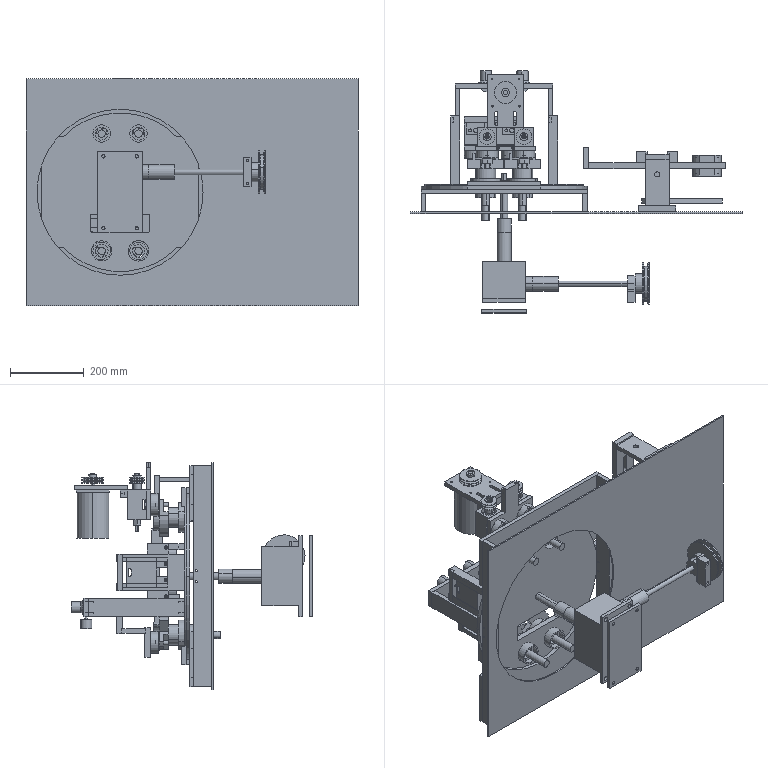Assembly | SolidWorks | mm | 86 component files | 87 solids | 1942 faces | box 900 x 656 x 616.29 mm | volume 16364994 mm3 | cylinder 1056 | plane 736 | cone 150 | commonest cylinder face diameters 5 x140 6.8 x104 7 x102 11 x94 6.6 x82 12 x52 35 x34 15 x28
Bill of materials:
AdjustmentSupportPlate | 2 |  | Long, slender rectangular bar with two small holes drilled into one end face.
AdjustmentTopPlate | 1 |  | Flat rectangular bar or strip plate with six through holes: two larger holes near the middle and two smaller holes at each end.
AdjustmentWheel | 2 |  | Turned part with a short cylindrical shank and a larger head. The head has a short cylindrical rim and a conical taper down to the shank, and a small axial hole in its face.
Axis | 2 |  | Stepped, hollow cylindrical part with a central bore running the full length. It has several diameter steps, a larger collar with flats near one end, and a short, slightly tapered spigot at that end.
BearingHeighteningSeat | 1 |  | Rectangular block, tall compared with its width, with two through holes across its thinner dimension near each end.
BearingHousing1 | 2 |  | Tubular sleeve with a large through bore and a raised flange around its middle. The flange has three equally spaced through holes.
BearingHousing2 | 2 |  | Flanged bushing: a cylindrical hub with a wider flange at one end, a large central through bore, and three equally spaced holes in the flange.
BearingHousingMountingPlate | 2 |  | Long flat rectangular bar with through holes of different sizes: one small hole, one medium hole, and near one end a large hole surrounded by four small holes in a square pattern. Two holes are drilled into the end face nearest the large hole.
BevelGearPlate1 | 1 |  | Thick rectangular plate with many through holes: four in a row along one edge, two larger holes in the middle, and five along the opposite edge. A shallow step or groove runs along one long edge on one face.
BevelGearPlate2 | 2 |  | Solid rectangular block with three vertical through holes in a row: a larger centre hole between two smaller holes, offset toward one long side.
BrassGuideRail | 2 |  | Thick rectangular plate with an undercut channel (T-slot-like profile) along one edge, four blind holes with conical bottoms, and one central through hole on the main face.
CenterAxis | 1 |  | Solid stepped round shaft: a long main diameter, a reduced-diameter section at one end, and two successive smaller steps at the other end.
Coupling1 | 1 |  | Thick-walled cylindrical sleeve with a central through bore that has a single rectangular keyway, plus two small holes on the outer cylindrical surface near each end.
Coupling2 | 1 |  | Solid cylindrical hub or sleeve with a smaller central through bore that has one rectangular keyway; plain outer surface.
CouplingAxis | 4 |  | Solid stepped round shaft or pin with four coaxial diameter sections: a long small-diameter end, a short largest-diameter collar, a middle step, and a slightly smaller end section.
CouplingPlate | 1 |  | Flat inverted-T plate: a wide rectangular base with a narrower rectangular tab rising from its center. The base has two large circular through holes, each surrounded by eight small holes on a bolt circle. Two small holes go into the top edge of the tab.
Disc | 1 |  | Thin circular disc with four large circular through holes (two near the top, two slightly larger near the bottom), a small central hole, and a rounded-corner rectangular slot below the center. The edge views show a slight step around the rim.
DiscBasePlate | 1 |  | Two separate thin rectangular plates under a single ID, placed mirrored with a gap between them. Each has a large circular-arc cutout on its inner long edge, so together they outline a circular opening. Each plate has small holes near its corners and near the ends of the arc.
DiscLimitPlate | 2 |  | Thick rectangular bar with a shallow concave circular-arc cut along one long edge, so it is narrowest at mid-length. There are two through holes near the ends along the straight edge.
DiscLimitPlateBasePlate | 2 |  | Straight rectangular bar with two circular through holes, one near each end, through the narrow dimension.
HolePunchingCouplingBushing | 1 |  | Plain thick-walled cylindrical tube or spacer with a concentric round through bore, about as long as its diameter.
Die | 2 |  | Rectangular block with an obround slot through its thickness near one edge, and a narrow channel running from that edge into the slot.
LocatingDieAdjustmentBlock | 2 |  | Elongated stepped block: a thinner full-length flange plate with a small hole at each end, joined to a thicker shorter central body. A larger circular through hole passes through the middle.
LocatingDieHolder | 2 |  | U-shaped (C-shaped) flat frame plate: a solid back section with two parallel arms around a large rectangular opening that is open at one end. Small rectangular notches cut into one face near the free ends of the arms.
LockingWheel | 2 |  | Coaxial stepped cylinder: a large short cylindrical base, then a short medium-diameter step, then a long slender pin.
LowerRollerFixingRing | 4 |  | Thick circular disc with a large central through hole and four smaller through holes evenly spaced on a circle around it.
Motor | 1 |  | Cylindrical body topped by a thin square plate with four corner holes, and a slender cylindrical shaft sticking out of the plate's centre.
Motor2 | 1 |  | Rectangular box-shaped body with a thin rectangular flange plate on one face that has four corner holes. A cylindrical boss with a smaller shaft sticks out of a side face.
MotorMount | 1 |  | Flat rectangular plate with one large round through hole, four small round holes arranged in a rectangle, and two parallel elongated slots.
MotorMount2 | 1 |  | Thin flat rectangular plate with four small round through holes near the corners.
MotorPlateFixingBlock | 1 |  | Rectangular bar block with two larger through holes along one axis, through the side faces, and two smaller through holes at right angles to them, through the top face.
MotorPulley | 1 |  | Round grooved wheel with two V-shaped circumferential grooves, a raised cylindrical hub on one face, a central through bore, and small radial holes in the hub.
p002 | 1 |  | Extruded profile part: a straight rectangular bar with a lug off one side that has a semicircular end and a round through hole.
Panel | 1 |  | Very thin rectangular sheet with one large circular hole set toward one end.
PunchingAxisSeat | 2 |  | Rectangular block with a large stepped/counterbored round bore from the top, a rectangular notch or slot cut across one side, and four round holes in a side face.
RearRoller | 2 |  | Shaft with a disc on one end. The disc has a wedge-shaped sector cut out, and a narrower arm with a round hole extends into that cut-out area. A short cylindrical boss is on the opposite face.
ReducerCoupling | 1 |  | Long slender stepped cylindrical shaft: larger-diameter central body with a shorter, reduced-diameter journal at each end.
ReducerPulley | 1 |  | Single-groove sheave/pulley-like disc with a cylindrical hub on one side and a central bore with a keyway notch.
Roller | 2 |  | Semicircular (half-disc) body with a rectangular upright tab that has a round hole, a long cylindrical pin sticking out of one face, and a short cylindrical boss on the opposite face.
SmallPulley | 2 |  | Double-groove V-pulley-like body with three flanges forming two V-grooves, a cylindrical hub extending on both sides, and a keyed central bore.
SpringPullPlate | 1 |  | Flat L-shaped plate of constant thickness with four through-holes: one larger and two small holes in the short leg, and one medium hole near the end of the long leg.
SpringPullPlateFixingAxis | 1 |  | Stepped cylindrical pin: a short larger-diameter cylindrical head with a longer, smaller-diameter plain shank.
SupportPlate_2 | 1 |  | Thick rectangular plate with two large circular through-bores. Each bore is surrounded by four small holes in a square pattern, and a row of five holes runs along the upper edge. One edge has a rectangular step or rebate.
SupportPlate | 2 |  | Long, thin rectangular bar or strip with a few small holes on its narrow faces: pairs near each end on one face and two holes near mid-length on the adjacent face.
SupportPlate2 | 1 |  | Rectangular flat plate or block with five evenly spaced round holes drilled into one long edge face.
TractionBasePlate | 1 |  | Long, flat rectangular plate with four corner holes, two pairs of smaller holes (one pair near each end region), and one single hole lower down the centreline.
TractionBearingHousing | 4 |  | Round flange with two parallel flats, a large central bore, four through-holes at the corners, and a raised annular pilot boss on one face.
TractionHandwheelAdjustmentPlate | 1 |  | Solid rectangular block with one round through-hole perpendicular to its largest face.
TractionSmallCylinderSeat | 1 |  | Plain rectangular block with a roughly square footprint. Its height is less than its width. No holes, cutouts, chamfers or other features are visible.
TractionTensionPlate | 2 |  | Thick rectangular plate, close to square in face view. It has two round through-holes lined up along one edge and one horizontal obround (slotted) through-hole near the opposite edge.
TractionUpperPlate | 1 |  | Long, narrow, thin flat bar. Along its centerline it has three elongated through-slots of different lengths and widths, plus one larger round hole near one end. It also has four small round holes, two near each end.
TractionVerticalPlate | 2 |  | Rectangular flat plate with one round hole through the top face, set off-center toward one end. Two smaller round holes are drilled into one long side face.
TurntableFixingNut | 4 |  | Cylindrical sleeve or bushing with a concentric round central bore through its length. Four evenly spaced rectangular notches run lengthwise along the full length of the outer surface.
Mates:
1. coincident | Panel-1 face at (-419.784, 370.983, 311.5) dir (0, 1, 0) | SupportPlate-1 face at (-389.784, 370.983, 304) dir (0, -1, 0)
2. concentric | DiscBasePlate-1 face at (-164.784, 430.983, 4) dir (0, -1, 0) r 215 | Panel-1 face at (-164.784, 370.983, 4) dir (0, -1, 0) r 225
3. distance | DiscBasePlate-1 face at (-164.784, 420.983, 4) dir (0, -1, 0) | Panel-1 face at (-419.784, 370.983, 311.5) dir (0, 1, 0)
4. coincident | DiscBasePlate-1 face at (-389.784, 430.983, 154) dir (-1, 0, 0) | SupportPlate-1 face at (-389.784, 420.983, 304) dir (-1, 0, 0)
5. coincident | DiscBasePlate-1 face at (60.216, 430.983, 304) dir (0, 0, 1) | SupportPlate-1 face at (-389.784, 370.983, 304) dir (0, 0, 1)
6. coincident | DiscBasePlate-1 face at (60.216, 430.983, 304) dir (0, 0, 1) | SupportPlate-2 face at (48.216, 370.983, 304) dir (0, 0, 1)
7. coincident | DiscBasePlate-1 face at (60.216, 430.983, 154) dir (1, 0, 0) | SupportPlate-2 face at (60.216, 420.983, 304) dir (1, 0, 0)
8. coincident | Panel-1 face at (-419.784, 370.983, 311.5) dir (0, 1, 0) | SupportPlate-2 face at (48.216, 370.983, 304) dir (0, -1, 0)
9. concentric | DiscBasePlate-1 face at (-164.784, 430.983, 4) dir (0, -1, 0) r 215 | Disc-1 face at (-164.784, 445.983, 4) dir (0, -1, 0) r 225
10. coincident | Disc-1 face at (-164.784, 430.983, 4) dir (0, -1, 0) | DiscBasePlate-1 face at (-164.784, 430.983, 4) dir (0, 1, 0)
11. parallel | DiscBasePlate-1 face at (60.216, 430.983, -296) dir (0, 0, -1) | Disc-1 face at (-239.784, 445.983, -105.5) dir (0, 0, 1)
12. concentric | Disc-1 face at (-164.784, 440.983, 4) dir (0, 1, 0) r 215 | DiscLimitPlate-1 face at (-164.784, 452.983, 4) dir (0, -1, 0) r 215
13. coincident | DiscLimitPlate-1 face at (-164.784, 440.983, 4) dir (0, -1, 0) | Disc-1 face at (-164.784, 440.983, 4) dir (0, 1, 0)
14. parallel | DiscBasePlate-1 face at (60.216, 430.983, 304) dir (0, 0, 1) | DiscLimitPlate-1 face at (-264.784, 452.983, 244.329) dir (0, 0, 1)
15. coincident | DiscBasePlate-1 face at (-164.784, 430.983, 4) dir (0, 1, 0) | DiscLimitPlateBasePlate-1 face at (-264.784, 430.983, 229.329) dir (0, -1, 0)
16. coincident | DiscLimitPlate-1 face at (-264.784, 452.983, 194.329) dir (-1, 0, 0) | DiscLimitPlateBasePlate-1 face at (-264.784, 430.983, 244.329) dir (-1, 0, 0)
17. coincident | DiscLimitPlate-1 face at (-264.784, 452.983, 244.329) dir (0, 0, 1) | DiscLimitPlateBasePlate-1 face at (-264.784, 430.983, 244.329) dir (0, 0, 1)
18. concentric | Disc-1 face at (-164.784, 440.983, 4) dir (0, 1, 0) r 215 | DiscLimitPlate-2 face at (-164.784, 452.983, 4) dir (0, -1, 0) r 215
19. parallel | DiscBasePlate-1 face at (60.216, 430.983, -296) dir (0, 0, -1) | DiscLimitPlate-2 face at (-64.784, 452.983, -236.329) dir (0, 0, -1)
20. coincident | DiscLimitPlate-2 face at (-164.784, 440.983, 4) dir (0, -1, 0) | Disc-1 face at (-164.784, 440.983, 4) dir (0, 1, 0)
21. coincident | DiscBasePlate-1 face at (-164.784, 430.983, 4) dir (0, 1, 0) | DiscLimitPlateBasePlate-2 face at (-264.784, 430.983, -221.329) dir (0, -1, 0)
22. coincident | DiscLimitPlate-2 face at (-64.784, 452.983, -186.329) dir (1, 0, 0) | DiscLimitPlateBasePlate-2 face at (-64.784, 440.983, -236.329) dir (1, 0, 0)
23. coincident | DiscLimitPlate-2 face at (-64.784, 452.983, -236.329) dir (0, 0, -1) | DiscLimitPlateBasePlate-2 face at (-264.784, 440.983, -236.329) dir (0, 0, -1)
24. coincident | Disc-1 face at (-164.784, 445.983, 4) dir (0, 1, 0) | AdjustmentSupportPlate-1 face at (-285.284, 445.983, -105.5) dir (0, -1, 0)
25. parallel | Disc-1 face at (-84.784, 445.983, -100.5) dir (-1, 0, 0) | AdjustmentSupportPlate-1 face at (-285.284, 705.983, -55.5) dir (1, 0, 0)
26. coincident | Disc-1 face at (-239.784, 445.983, -105.5) dir (0, 0, 1) | AdjustmentSupportPlate-1 face at (-285.284, 705.983, -105.5) dir (0, 0, -1)
27. coincident | Disc-1 face at (-164.784, 445.983, 4) dir (0, 1, 0) | AdjustmentSupportPlate-2 face at (-32.284, 445.983, -55.5) dir (0, -1, 0)
28. coincident | AdjustmentSupportPlate-1 face at (-285.284, 705.983, -55.5) dir (0, 0, 1) | AdjustmentSupportPlate-2 face at (-32.284, 445.983, -55.5) dir (0, 0, 1)
29. distance | AdjustmentSupportPlate-2 face at (-32.284, 445.983, -105.5) dir (1, 0, 0) | AdjustmentSupportPlate-1 face at (-297.284, 705.983, -55.5) dir (-1, 0, 0)
30. coincident | AdjustmentTopPlate-1 face at (-297.284, 705.983, -105.5) dir (0, -1, 0) | AdjustmentSupportPlate-1 face at (-285.284, 705.983, -105.5) dir (0, 1, 0)
31. coincident | AdjustmentTopPlate-1 face at (-297.284, 705.983, -55.5) dir (-1, 0, 0) | AdjustmentSupportPlate-1 face at (-297.284, 705.983, -55.5) dir (-1, 0, 0)
32. coincident | AdjustmentTopPlate-1 face at (-297.284, 705.983, -55.5) dir (0, 0, 1) | AdjustmentSupportPlate-1 face at (-285.284, 705.983, -55.5) dir (0, 0, 1)
33. distance | Disc-1 face at (-244.784, 445.983, -60.5) dir (1, 0, 0) | AdjustmentSupportPlate-1 face at (-285.284, 705.983, -55.5) dir (1, 0, 0)
34. concentric | Disc-1 edge at (-214.784, 445.983, 163) dir (0, -1, 0) r 23.5 | BearingHousing2-1 face at (-214.784, 440.309, 163) dir (0, -1, 0) r 40
35. coincident | Disc-1 face at (-164.784, 445.983, 4) dir (0, 1, 0) | BearingHousing2-1 face at (-250.623, 445.983, 180.764) dir (0, -1, 0)
36. concentric | Disc-1 face at (-214.784, 445.983, -155) dir (0, -1, 0) r 27.5 | BearingHousing1-1 face at (-214.784, 440.309, -155) dir (0, -1, 0) r 27.5
37. coincident | Disc-1 face at (-164.784, 445.983, 4) dir (0, 1, 0) | BearingHousing1-1 face at (-249.957, 445.983, -174.049) dir (0, -1, 0)
38. concentric | Disc-1 face at (-114.784, 445.983, 163) dir (0, -1, 0) r 23.5 | BearingHousing2-2 face at (-114.784, 440.309, 163) dir (0, -1, 0) r 40
39. coincident | Disc-1 face at (-164.784, 445.983, 4) dir (0, 1, 0) | BearingHousing2-2 face at (-150.95, 445.983, 145.912) dir (0, -1, 0)
40. concentric | Disc-1 face at (-114.784, 445.983, -155) dir (0, -1, 0) r 27.5 | BearingHousing1-2 face at (-114.784, 440.309, -155) dir (0, -1, 0) r 27.5
41. coincident | Disc-1 face at (-164.784, 445.983, 4) dir (0, 1, 0) | BearingHousing1-2 face at (-142.56, 445.983, -183.783) dir (0, -1, 0)
42. concentric | BearingHousing1-2 face at (-114.784, 440.309, -155) dir (0, -1, 0) r 17.5 | RearRoller-3 face at (-114.784, 404.838, -155) dir (0, -1, 0) r 10
43. concentric | BearingHousing1-1 face at (-214.784, 440.309, -155) dir (0, -1, 0) r 17.5 | RearRoller-4 face at (-214.784, 404.838, -155) dir (0, -1, 0) r 10
44. parallel | RearRoller-3 face at (-151.129, 348.983, -199.045) dir (0.6062, 0, -0.7953) | RearRoller-4 face at (-251.129, 348.983, -199.045) dir (0.6062, 0, -0.7953)
45. coincident | RearRoller-3 face at (-93.568, 513.983, -182.837) dir (0, 1, 0) | RearRoller-4 face at (-193.568, 513.983, -182.837) dir (0, 1, 0)
46. concentric | BearingHousing2-1 face at (-214.784, 440.309, 163) dir (0, -1, 0) r 17.5 | Roller-5 face at (-214.784, 444.838, 163) dir (0, -1, 0) r 10
47. coincident | BearingHousing2-1 face at (-235.839, 488.983, 173.436) dir (0, 1, 0) | Roller-5 face at (-264.482, 488.983, 168.486) dir (0, -1, 0)
48. concentric | BearingHousing2-2 face at (-114.784, 440.309, 163) dir (0, -1, 0) r 17.5 | Roller-6 face at (-114.784, 444.838, 163) dir (0, -1, 0) r 10
49. coincident | BearingHousing2-2 face at (-136.031, 488.983, 152.961) dir (0, 1, 0) | Roller-6 face at (-164.482, 488.983, 168.486) dir (0, -1, 0)
50. parallel | Roller-5 face at (-195.761, 388.983, 216.843) dir (0.994, 0, -0.1097) | Roller-6 face at (-95.761, 388.983, 216.843) dir (0.994, 0, -0.1097)
51. coincident | RearRoller-3 face at (-84.476, 488.983, -194.767) dir (0, -1, 0) | RearRoller-4 face at (-184.476, 488.983, -194.767) dir (0, -1, 0)
52. coincident | BearingHousing1-1 face at (-235.448, 488.983, -166.191) dir (0, 1, 0) | RearRoller-4 face at (-184.476, 488.983, -194.767) dir (0, -1, 0)
53. concentric | Roller-5 face at (-210.944, 388.983, 197.789) dir (0, 1, 0) r 6 | CouplingAxis-1 face at (-210.944, 520.733, 197.789) dir (0, 1, 0) r 6
54. concentric | LowerRollerFixingRing-1 face at (-210.944, 542.523, 197.789) dir (0, 1, 0) r 10 | CouplingAxis-1 face at (-210.944, 520.733, 197.789) dir (0, 1, 0) r 6
55. coincident | LowerRollerFixingRing-1 face at (-193.444, 525.983, 197.789) dir (0, 1, 0) | CouplingAxis-1 edge at (-210.944, 525.983, 197.789) dir (0, 1, 0) r 7.5
56. concentric | CouplingPlate-1 face at (-210.944, 548.983, 197.789) dir (0, -1, 0) r 17.5 | CouplingAxis-1 face at (-210.944, 520.733, 197.789) dir (0, 1, 0) r 7
57. parallel | DiscLimitPlateBasePlate-1 face at (-264.784, 430.983, 244.329) dir (0, 0, 1) | CouplingPlate-1 face at (-135.944, 548.983, 312.789) dir (0, 0, 1)
58. concentric | CouplingPlate-1 face at (-210.944, 548.983, 220.789) dir (0, 1, 0) r 2.5 | LowerRollerFixingRing-1 face at (-210.944, 516.983, 220.789) dir (0, -1, 0) r 3.3
59. concentric | CouplingPlate-1 face at (-233.944, 548.983, 197.789) dir (0, 1, 0) r 2.5 | LowerRollerFixingRing-1 face at (-233.944, 516.983, 197.789) dir (0, -1, 0) r 3.3
60. coincident | CouplingPlate-1 face at (-79.944, 536.983, 237.789) dir (0, -1, 0) | LowerRollerFixingRing-1 face at (-180.944, 536.983, 197.789) dir (0, 1, 0)
61. coincident | Roller-5 face at (-249.572, 513.983, 166.84) dir (0, 1, 0) | CouplingAxis-1 face at (-215.967, 513.983, 194.507) dir (0, -1, 0)
62. concentric | CouplingPlate-1 face at (-110.944, 548.983, 197.789) dir (0, -1, 0) r 17.5 | CouplingAxis-2 face at (-110.944, 520.733, 197.789) dir (0, 1, 0) r 7
63. concentric | CouplingPlate-1 face at (-110.944, 548.983, 197.789) dir (0, -1, 0) r 17.5 | LowerRollerFixingRing-2 face at (-110.944, 542.523, 197.789) dir (0, 1, 0) r 17.5
64. coincident | CouplingPlate-1 face at (-79.944, 536.983, 237.789) dir (0, -1, 0) | LowerRollerFixingRing-2 face at (-80.944, 536.983, 197.789) dir (0, 1, 0)
65. concentric | CouplingPlate-1 face at (-110.944, 548.983, 220.789) dir (0, 1, 0) r 2.5 | LowerRollerFixingRing-2 face at (-110.944, 516.983, 220.789) dir (0, -1, 0) r 5.5
66. coincident | Roller-6 face at (-149.572, 513.983, 166.84) dir (0, 1, 0) | CouplingAxis-2 face at (-113.911, 513.983, 192.574) dir (0, -1, 0)
67. coincident | CouplingPlate-1 face at (-241.944, 548.983, 157.789) dir (0, 0, -1) | PunchingAxisSeat-1 face at (-185.944, 598.983, 157.789) dir (0, 0, -1)
68. coincident | CouplingPlate-1 face at (-79.944, 548.983, 237.789) dir (0, 1, 0) | PunchingAxisSeat-1 face at (-185.944, 548.983, 237.789) dir (0, -1, 0)
69. concentric | CouplingPlate-1 edge at (-226.944, 548.983, 217.789) dir (0, 1, 0) r 2.5 | PunchingAxisSeat-1 edge at (-226.944, 598.983, 217.789) dir (0, 1, 0) r 3.5
70. coincident | CouplingPlate-1 face at (-79.944, 548.983, 237.789) dir (0, 0, 1) | PunchingAxisSeat-2 face at (-85.944, 598.983, 237.789) dir (0, 0, 1)
71. coincident | CouplingPlate-1 face at (-79.944, 548.983, 237.789) dir (0, 1, 0) | PunchingAxisSeat-2 face at (-85.944, 548.983, 237.789) dir (0, -1, 0)
72. concentric | CouplingPlate-1 edge at (-94.944, 548.983, 177.789) dir (0, 1, 0) r 2.5 | PunchingAxisSeat-2 face at (-94.944, 548.983, 177.789) dir (0, 1, 0) r 3.5
73. coincident | MotorPlateFixingBlock-1 face at (-110.944, 598.983, 217.789) dir (0, -1, 0) | PunchingAxisSeat-2 face at (-85.944, 598.983, 237.789) dir (0, 1, 0)
74. concentric | CouplingAxis-3 face at (-242.621, 520.733, -176.215) dir (0, 1, 0) r 6 | LowerRollerFixingRing-4 face at (-242.621, 542.523, -176.215) dir (0, 1, 0) r 10
75. coincident | CouplingAxis-3 face at (-233.626, 525.983, -175.907) dir (0, 1, 0) | LowerRollerFixingRing-4 face at (-260.013, 525.983, -174.275) dir (0, 1, 0)
76. concentric | RearRoller-4 face at (-242.621, 348.983, -176.215) dir (0, 1, 0) r 6 | CouplingAxis-3 face at (-242.621, 520.733, -176.215) dir (0, 1, 0) r 6
77. coincident | RearRoller-4 face at (-193.568, 513.983, -182.837) dir (0, 1, 0) | CouplingAxis-3 face at (-236.624, 513.983, -176.01) dir (0, -1, 0)
78. coincident | LowerRollerFixingRing-5 face at (-154.995, 525.983, -163.841) dir (0, 1, 0) | CouplingAxis-5 face at (-134.193, 525.983, -173.059) dir (0, 1, 0)
79. concentric | LowerRollerFixingRing-5 face at (-142.621, 542.523, -176.215) dir (0, 1, 0) r 17.5 | CouplingAxis-5 face at (-142.621, 520.733, -176.215) dir (0, 1, 0) r 7
80. concentric | RearRoller-3 face at (-142.621, 348.983, -176.215) dir (0, 1, 0) r 6 | CouplingAxis-5 face at (-142.621, 520.733, -176.215) dir (0, 1, 0) r 6
81. coincident | RearRoller-3 face at (-93.568, 513.983, -182.837) dir (0, 1, 0) | CouplingAxis-5 face at (-137.002, 513.983, -174.111) dir (0, -1, 0)
82. coincident | LowerRollerFixingRing-4 face at (-272.436, 536.983, -172.888) dir (0, 1, 0) | SupportPlate_2-1 face at (-112.621, 536.983, -216.215) dir (0, -1, 0)
83. concentric | SupportPlate_2-1 face at (-242.621, 552.983, -176.215) dir (0, -1, 0) r 17.5 | CouplingAxis-3 face at (-242.621, 520.733, -176.215) dir (0, 1, 0) r 7
84. concentric | LowerRollerFixingRing-5 face at (-126.357, 516.983, -192.479) dir (0, -1, 0) r 3.3 | SupportPlate_2-1 edge at (-126.357, 552.983, -192.479) dir (0, 1, 0) r 2.5
85. concentric | SupportPlate_2-1 edge at (-252.621, 550.983, -144.215) dir (0, 1, 0) r 3.3 | SupportPlate2-3 edge at (-252.621, 550.983, -144.215) dir (0, -1, 0) r 3.4
86. concentric | SupportPlate_2-1 edge at (-132.621, 550.983, -144.215) dir (0, 1, 0) r 3.3 | SupportPlate2-3 edge at (-132.621, 550.983, -144.215) dir (0, -1, 0) r 3.4
87. parallel | SupportPlate2-3 face at (-272.621, 614.983, -138.215) dir (0, 1, 0) | BevelGearPlate1-2 face at (-112.621, 614.983, -138.215) dir (0, -1, 0)
88. concentric | SupportPlate2-3 face at (-132.621, 614.983, -144.215) dir (0, 1, 0) r 3.4 | BevelGearPlate1-2 edge at (-132.621, 628.983, -144.215) dir (0, -1, 0) r 3.5
89. concentric | SupportPlate2-3 face at (-132.621, 614.983, -144.215) dir (0, 1, 0) r 3.4 | BevelGearPlate1-2 edge at (-132.621, 628.983, -144.215) dir (0, -1, 0) r 3.5
90. concentric | SupportPlate2-3 face at (-252.621, 614.983, -144.215) dir (0, 1, 0) r 3.4 | BevelGearPlate1-2 face at (-252.621, 612.983, -144.215) dir (0, 1, 0) r 3.5
91. coincident | SupportPlate2-3 face at (-272.621, 614.983, -138.215) dir (0, 1, 0) | BevelGearPlate1-2 edge at (-112.621, 614.983, -150.215) dir (0, 0, 1)
92. concentric | SupportPlate_2-1 face at (-142.621, 552.983, -176.215) dir (0, -1, 0) r 17.5 | LowerRollerFixingRing-5 edge at (-142.621, 536.983, -176.215) dir (0, 1, 0) r 17.5
93. concentric | SupportPlate_2-1 face at (-126.357, 552.983, -192.479) dir (0, 1, 0) r 2.5 | LowerRollerFixingRing-5 face at (-126.357, 516.983, -192.479) dir (0, -1, 0) r 5.5
94. concentric | BevelGearPlate1-2 face at (-257.621, 628.983, -79.715) dir (0, 1, 0) r 5.5 | BevelGearPlate2-1 face at (-257.621, 612.983, -79.715) dir (0, 1, 0) r 3.4
95. coincident | BevelGearPlate1-2 face at (-112.621, 612.983, -67.215) dir (0, -1, 0) | BevelGearPlate2-1 face at (-266.621, 612.983, -67.215) dir (0, 1, 0)
96. parallel | BevelGearPlate1-2 face at (-112.621, 612.983, -67.215) dir (0, 0, 1) | BevelGearPlate2-1 face at (-266.621, 580.983, -67.215) dir (0, 0, 1)
97. coincident | SupportPlate_2-1 face at (-112.621, 550.983, -150.215) dir (0, 1, 0) | SupportPlate2-3 face at (-272.621, 550.983, -138.215) dir (0, -1, 0)
98. concentric | BevelGearPlate1-2 face at (-159.621, 628.983, -79.715) dir (0, 1, 0) r 5.5 | BevelGearPlate2-2 face at (-159.621, 612.983, -79.715) dir (0, 1, 0) r 3.4
99. coincident | BevelGearPlate1-2 face at (-112.621, 612.983, -67.215) dir (0, 0, 1) | BevelGearPlate2-2 face at (-168.621, 580.983, -67.215) dir (0, 0, 1)
100. coincident | BevelGearPlate1-2 face at (-112.621, 612.983, -67.215) dir (0, -1, 0) | BevelGearPlate2-2 face at (-168.621, 612.983, -67.215) dir (0, 1, 0)
101. concentric | PunchingAxisSeat-1 face at (-210.944, 573.983, 237.789) dir (0, 0, -1) r 11 | Axis-1 face at (-210.944, 573.983, 177.508) dir (0, 0, 1) r 7
102. coincident | PunchingAxisSeat-1 face at (-185.944, 598.983, 157.789) dir (0, 0, -1) | Axis-1 face at (-219.435, 579.265, 157.789) dir (0, 0, 1)
103. concentric | PunchingAxisSeat-2 face at (-110.944, 573.983, 225.789) dir (0, 0, 1) r 20 | Axis-2 face at (-110.944, 573.983, 177.508) dir (0, 0, 1) r 7
104. coincident | PunchingAxisSeat-2 face at (-85.944, 598.983, 157.789) dir (0, 0, -1) | Axis-2 face at (-102.626, 579.535, 157.789) dir (0, 0, 1)
105. parallel | Axis-1 face at (-216.039, 577.152, 282.789) dir (0, 0, 1) | SmallPulley-1 face at (-189.444, 573.983, 255.789) dir (0, 0, -1)
106. coincident | PunchingAxisSeat-1 face at (-185.944, 598.983, 237.789) dir (0, 0, 1) | SmallPulley-1 face at (-199.944, 573.983, 237.789) dir (0, 0, -1)
107. concentric | Axis-1 face at (-210.944, 573.983, 177.508) dir (0, 0, 1) r 6 | SmallPulley-1 face at (-210.944, 573.983, 228.868) dir (0, 0, -1) r 11
108. coincident | PunchingAxisSeat-2 face at (-85.944, 598.983, 237.789) dir (0, 0, 1) | SmallPulley-2 face at (-99.944, 573.983, 237.789) dir (0, 0, -1)
109. concentric | Axis-2 face at (-110.944, 573.983, 177.508) dir (0, 0, 1) r 6 | SmallPulley-2 face at (-110.944, 573.983, 228.868) dir (0, 0, -1) r 6
110. coincident | MotorPlateFixingBlock-1 face at (-110.944, 618.983, 237.789) dir (0, 0, 1) | PunchingAxisSeat-1 face at (-185.944, 598.983, 237.789) dir (0, 0, 1)
111. distance | MotorPlateFixingBlock-1 face at (-110.944, 618.983, 237.789) dir (1, 0, 0) | PunchingAxisSeat-2 face at (-85.944, 548.983, 237.789) dir (1, 0, 0)
112. coincident | MotorPlateFixingBlock-1 face at (-110.944, 618.983, 237.789) dir (0, 0, 1) | PunchingAxisSeat-2 face at (-85.944, 598.983, 237.789) dir (0, 0, 1)
113. concentric | MotorPlateFixingBlock-1 face at (-135.944, 608.983, 237.789) dir (0, 0, 1) r 3.4 | MotorMount-2 face at (-135.944, 608.983, 249.789) dir (0, 0, -1) r 4.5
114. concentric | MotorPlateFixingBlock-1 face at (-185.944, 608.983, 237.789) dir (0, 0, 1) r 3.4 | MotorMount-2 face at (-185.944, 608.983, 249.789) dir (0, 0, -1) r 4.5
115. concentric | Motor-1 face at (-160.944, 693.983, 281.789) dir (0, 0, -1) r 5.75 | MotorMount-2 face at (-160.944, 693.983, 249.789) dir (0, 0, -1) r 15
116. concentric | Motor-1 edge at (-124.194, 730.733, 237.789) dir (0, 0, -1) r 3.5 | MotorMount-2 edge at (-124.194, 730.733, 249.789) dir (0, 0, 1) r 2.5
117. coincident | Motor-1 face at (-115.944, 648.983, 237.789) dir (0, 0, 1) | MotorMount-2 face at (-210.944, 598.983, 237.789) dir (0, 0, -1)
118. coincident | MotorPlateFixingBlock-1 face at (-110.944, 618.983, 237.789) dir (0, 0, 1) | MotorMount-2 face at (-210.944, 598.983, 237.789) dir (0, 0, -1)
119. concentric | MotorPulley-1 edge at (-160.944, 693.983, 255.789) dir (0, 0, -1) r 6 | Motor-1 face at (-160.944, 693.983, 281.789) dir (0, 0, -1) r 5.75
120. coincident | SmallPulley-1 face at (-199.944, 573.983, 272.789) dir (0, 0, 1) | MotorPulley-1 face at (-149.944, 693.983, 272.789) dir (0, 0, 1)
121. coincident | LowerRollerFixingRing-2 face at (-80.944, 536.983, 197.789) dir (0, 1, 0) | TurntableFixingNut-1 face at (-110.944, 536.983, 197.789) dir (0, -1, 0)
122. concentric | CouplingAxis-2 face at (-110.944, 520.733, 197.789) dir (0, 1, 0) r 7 | TurntableFixingNut-1 face at (-110.944, 554.983, 197.789) dir (0, 1, 0) r 7
123. coincident | LowerRollerFixingRing-1 face at (-180.944, 536.983, 197.789) dir (0, 1, 0) | TurntableFixingNut-4 face at (-210.944, 536.983, 197.789) dir (0, -1, 0)
124. concentric | CouplingAxis-1 face at (-210.944, 520.733, 197.789) dir (0, 1, 0) r 7 | TurntableFixingNut-4 face at (-210.944, 554.983, 197.789) dir (0, 1, 0) r 7
125. coincident | LowerRollerFixingRing-5 face at (-163.834, 536.983, -155.002) dir (0, 1, 0) | TurntableFixingNut-5 face at (-142.621, 536.983, -176.215) dir (0, -1, 0)
126. concentric | CouplingAxis-5 face at (-142.621, 520.733, -176.215) dir (0, 1, 0) r 7 | TurntableFixingNut-5 face at (-142.621, 554.983, -176.215) dir (0, 1, 0) r 7
127. coincident | LowerRollerFixingRing-4 face at (-272.436, 536.983, -172.888) dir (0, 1, 0) | TurntableFixingNut-6 face at (-242.621, 536.983, -176.215) dir (0, -1, 0)
128. concentric | CouplingAxis-3 face at (-242.621, 520.733, -176.215) dir (0, 1, 0) r 7 | TurntableFixingNut-6 face at (-242.621, 554.983, -176.215) dir (0, 1, 0) r 7
129. concentric | Motor2-1 face at (-164.784, 275.983, 4) dir (0, -1, 0) r 8.5 | Disc-1 face at (-164.784, 445.983, 4) dir (0, -1, 0) r 10
130. concentric | MotorMount2-1 edge at (-209.784, 106.983, -93.896) dir (0, 1, 0) r 4.4 | Motor2-1 edge at (-209.784, 135.983, -93.896) dir (0, 1, 0) r 6
131. concentric | MotorMount2-1 edge at (-119.784, 106.983, -93.896) dir (0, 1, 0) r 4.4 | Motor2-1 edge at (-119.784, 135.983, -93.896) dir (0, 1, 0) r 6
132. coincident | Disc-1 face at (-164.784, 445.983, 4) dir (0, 1, 0) | LocatingDie-1/LocatingDieHolder-1 face at (-44.284, 445.983, -36) dir (0, -1, 0)
133. parallel | AdjustmentSupportPlate-2 face at (-32.284, 445.983, -105.5) dir (1, 0, 0) | LocatingDie-1/LocatingDieHolder-1 face at (-19.284, 445.983, -36) dir (1, 0, 0)
134. coincident | AdjustmentSupportPlate-2 face at (-44.284, 445.983, -105.5) dir (-1, 0, 0) | LocatingDie-1/LocatingDieHolder-1 face at (-44.284, 445.983, -36) dir (-1, 0, 0)
135. distance | LocatingDie-1/LocatingDieHolder-1 face at (-44.284, 630.983, -36) dir (0, 0, -1) | DiscBasePlate-1 face at (60.216, 430.983, -296) dir (0, 0, -1)
136. concentric | Motor2-1 face at (-164.784, 275.983, 4) dir (0, -1, 0) r 8.5 | Coupling1-1 face at (-164.784, 315.983, 4) dir (0, -1, 0) r 8.5
137. coincident | Motor2-1 face at (-107.284, 235.983, 84) dir (0, 1, 0) | Coupling1-1 face at (-164.784, 235.983, 4) dir (0, -1, 0)
138. concentric | Coupling1-1 face at (-164.784, 315.983, 4) dir (0, -1, 0) r 8.5 | CenterAxis-1 face at (-164.784, 362.063, 4) dir (0, 1, 0) r 6
139. coincident | Coupling1-1 face at (-164.784, 315.983, 4) dir (0, 1, 0) | CenterAxis-1 face at (-172.84, 315.983, 1.29) dir (0, -1, 0)
140. coincident | BearingHeighteningSeat-1 face at (190.216, 153.983, 18.736) dir (1, 0, 0) | p002-2 face at (190.216, 175.983, 58.736) dir (1, 0, 0)
141. concentric | Motor2-1 face at (-57.284, 175.983, 58.736) dir (-1, 0, 0) r 6 | p002-2 edge at (190.216, 175.983, 58.736) dir (1, 0, 0) r 7.5
142. coincident | BearingHeighteningSeat-1 face at (170.216, 153.983, 18.736) dir (0, 1, 0) | p002-2 face at (190.216, 153.983, 98.736) dir (0, -1, 0)
143. coincident | BearingHeighteningSeat-1 face at (190.216, 153.983, 18.736) dir (0, 0, -1) | p002-2 face at (190.216, 160.983, 18.736) dir (0, 0, -1)
144. coincident | Motor2-1 face at (-87.284, 175.983, 58.736) dir (1, 0, 0) | Coupling2-1 face at (-87.284, 175.983, 58.736) dir (-1, 0, 0)
145. coincident | Motor2-1 face at (-57.284, 175.983, 58.736) dir (-1, 0, 0) r 6 | Coupling2-1 edge at (-17.284, 175.983, 58.736) dir (1, 0, 0) r 6
146. coincident | Coupling2-1 face at (-17.284, 175.983, 58.736) dir (1, 0, 0) | ReducerCoupling-1 face at (-17.284, 181.983, 58.736) dir (-1, 0, 0)
147. concentric | Coupling2-1 face at (-17.284, 175.983, 58.736) dir (-1, 0, 0) r 6 | ReducerCoupling-1 face at (52.758, 175.983, 58.736) dir (1, 0, 0) r 7.5
148. coincident | ReducerCoupling-1 face at (52.758, 175.983, 58.736) dir (1, 0, 0) r 6 | ReducerPulley-1 edge at (219.216, 175.983, 58.736) dir (-1, 0, 0) r 6
149. concentric | AdjustmentTopPlate-1 edge at (-214.784, 717.983, -80.5) dir (0, -1, 0) r 5 | AdjustmentWheel-1 face at (-214.784, 725.466, -80.5) dir (0, -1, 0) r 15
150. concentric | AdjustmentTopPlate-1 face at (-114.784, 717.983, -80.5) dir (0, -1, 0) r 5 | AdjustmentWheel-2 face at (-114.784, 725.466, -80.5) dir (0, -1, 0) r 15
151. coincident | AdjustmentTopPlate-1 face at (-297.284, 717.983, -105.5) dir (0, 1, 0) | AdjustmentWheel-2 face at (-134.69, 717.983, -82.43) dir (0, -1, 0)
152. coincident | AdjustmentTopPlate-1 face at (-297.284, 717.983, -105.5) dir (0, 1, 0) | AdjustmentWheel-1 face at (-234.69, 717.983, -82.43) dir (0, -1, 0)
153. concentric | AdjustmentTopPlate-1 face at (-214.784, 711.983, -105.5) dir (0, 0, -1) r 3.4 | LockingWheel-1 face at (-214.784, 711.983, -103.239) dir (0, 0, 1) r 3
154. coincident | AdjustmentTopPlate-1 face at (-297.284, 705.983, -105.5) dir (0, 0, -1) | LockingWheel-1 face at (-211.724, 713.682, -105.5) dir (0, 0, 1)
155. coincident | AdjustmentTopPlate-1 face at (-297.284, 705.983, -105.5) dir (0, 0, -1) | LockingWheel-2 face at (-111.284, 711.983, -105.5) dir (0, 0, 1)
156. concentric | AdjustmentTopPlate-1 face at (-114.784, 711.983, -105.5) dir (0, 0, -1) r 3.4 | LockingWheel-2 face at (-114.784, 711.983, -103.239) dir (0, 0, 1) r 3
157. coincident | TractionVerticalPlate-1 face at (217.716, 511.983, 272.5) dir (0, 1, 0) | TractionUpperPlate-2 face at (217.716, 511.983, 276.5) dir (0, -1, 0)
158. concentric | TractionVerticalPlate-3 face at (230.216, 511.983, -133.5) dir (0, 1, 0) r 2.5 | TractionUpperPlate-2 face at (230.216, 511.983, -133.5) dir (0, 1, 0) r 3.5
159. concentric | TractionVerticalPlate-3 face at (270.216, 511.983, -133.5) dir (0, 1, 0) r 2.5 | TractionUpperPlate-2 face at (270.216, 511.983, -133.5) dir (0, 1, 0) r 3.5
160. parallel | TractionVerticalPlate-1 face at (217.716, 386.983, 272.5) dir (0, 0, 1) | TractionUpperPlate-2 face at (282.716, 511.983, 276.5) dir (0, 0, 1)
161. concentric | BearingHousingMountingPlate-3 face at (385.216, 487.983, 59.606) dir (0, 1, 0) r 20 | TractionBearingHousing-1 face at (385.216, -501.017, 59.606) dir (0, -1, 0) r 20
162. coincident | BearingHousingMountingPlate-3 face at (65.216, 503.983, 27.106) dir (0, 1, 0) | TractionBearingHousing-1 face at (385.216, 503.983, 98.606) dir (0, -1, 0)
163. concentric | BearingHousingMountingPlate-2 face at (385.216, 487.983, -28.052) dir (0, 1, 0) r 20 | TractionBearingHousing-2 face at (385.216, -501.017, -28.052) dir (0, -1, 0) r 15
164. coincident | BearingHousingMountingPlate-3 face at (65.216, 487.983, 92.106) dir (0, 0, 1) | TractionBearingHousing-1 face at (422.075, 498.983, 92.106) dir (0, 0, 1)
165. coincident | BearingHousingMountingPlate-2 face at (65.216, 487.983, 4.448) dir (0, 0, 1) | TractionBearingHousing-2 face at (422.075, 498.983, 4.448) dir (0, 0, 1)
166. concentric | TractionBearingHousing-3 face at (385.216, 1492.983, 59.606) dir (0, 1, 0) r 23.5 | BearingHousingMountingPlate-3 face at (385.216, 487.983, 59.606) dir (0, 1, 0) r 20
167. coincident | TractionBearingHousing-3 face at (385.216, 487.983, 20.606) dir (0, 1, 0) | BearingHousingMountingPlate-3 face at (65.216, 487.983, 27.106) dir (0, -1, 0)
168. coincident | BearingHousingMountingPlate-3 face at (65.216, 487.983, 27.106) dir (0, 0, -1) | TractionBearingHousing-3 face at (422.075, 492.983, 27.106) dir (0, 0, -1)
169. concentric | BearingHousingMountingPlate-2 face at (385.216, 487.983, -28.052) dir (0, 1, 0) r 20 | TractionBearingHousing-6 edge at (385.216, 492.983, -28.052) dir (0, 1, 0) r 15
170. coincident | BearingHousingMountingPlate-2 face at (65.216, 487.983, -60.552) dir (0, -1, 0) | TractionBearingHousing-6 face at (385.216, 487.983, -67.052) dir (0, 1, 0)
171. concentric | TractionTensionPlate-1 face at (65.216, 495.983, -5.552) dir (-1, 0, 0) r 4.5 | BearingHousingMountingPlate-2 face at (65.216, 495.983, -5.552) dir (-1, 0, 0) r 3.4
172. concentric | BearingHousingMountingPlate-2 edge at (65.216, 495.983, -50.552) dir (-1, 0, 0) r 3.4 | TractionTensionPlate-1 face at (65.216, 495.983, -50.552) dir (-1, 0, 0) r 4.5
173. coincident | BearingHousingMountingPlate-2 face at (65.216, 487.983, 4.448) dir (-1, 0, 0) | TractionTensionPlate-1 face at (65.216, 487.983, 4.448) dir (1, 0, 0)
174. coincident | BearingHousingMountingPlate-3 face at (65.216, 487.983, 92.106) dir (-1, 0, 0) | TractionTensionPlate-2 face at (65.216, 487.983, 92.106) dir (1, 0, 0)
175. coincident | BearingHousingMountingPlate-3 face at (65.216, 487.983, 27.106) dir (0, -1, 0) | TractionTensionPlate-2 face at (65.216, 487.983, 92.106) dir (0, -1, 0)
176. coincident | TractionBearingHousing-2 face at (385.216, 503.983, 10.948) dir (0, -1, 0) | BearingHousingMountingPlate-2 face at (65.216, 503.983, -60.552) dir (0, 1, 0)
177. coincident | BearingHousingMountingPlate-3 face at (65.216, 487.983, 27.106) dir (0, 0, -1) | BrassGuideRail-3 face at (195.216, 503.983, 27.106) dir (0, 0, -1)
178. coincident | TractionUpperPlate-2 face at (217.716, 511.983, 276.5) dir (-1, 0, 0) | BrassGuideRail-3 face at (217.716, 527.983, 132.106) dir (1, 0, 0)
179. coincident | TractionUpperPlate-2 face at (217.716, 511.983, 276.5) dir (0, -1, 0) | BrassGuideRail-3 face at (217.716, 511.983, 132.106) dir (0, 1, 0)
180. coincident | BearingHousingMountingPlate-3 face at (65.216, 503.983, 27.106) dir (0, 1, 0) | BrassGuideRail-3 face at (195.216, 503.983, 132.106) dir (0, -1, 0)
181. coincident | BearingHousingMountingPlate-2 face at (65.216, 487.983, 4.448) dir (0, 0, 1) | BrassGuideRail-4 face at (305.216, 503.983, 4.448) dir (0, 0, 1)
182. concentric | BrassGuideRail-4 face at (250.216, 406.983, -28.052) dir (0, 1, 0) r 5.5 | BearingHousingMountingPlate-2 face at (250.216, 487.983, -28.052) dir (0, 1, 0) r 9.5
183. coincident | TractionUpperPlate-2 face at (217.716, 511.983, 276.5) dir (-1, 0, 0) | BrassGuideRail-4 face at (217.716, 527.983, -100.552) dir (1, 0, 0)
184. coincident | TractionUpperPlate-2 face at (217.716, 511.983, 276.5) dir (0, -1, 0) | BrassGuideRail-4 face at (282.716, 511.983, -100.552) dir (0, 1, 0)
185. coincident | BearingHousingMountingPlate-2 face at (65.216, 503.983, -60.552) dir (0, 1, 0) | BrassGuideRail-4 face at (305.216, 503.983, -100.552) dir (0, -1, 0)
186. coincident | Panel-1 face at (-419.784, 370.983, 311.5) dir (0, 1, 0) | TractionBasePlate-2 face at (300.216, 370.983, 301.5) dir (0, -1, 0)
187. distance | TractionBasePlate-2 face at (200.216, 386.983, 301.5) dir (0, 0, 1) | Panel-1 face at (-419.784, 370.983, 311.5) dir (0, 0, 1)
188. concentric | TractionVerticalPlate-1 edge at (270.216, 386.983, 266.5) dir (0, -1, 0) r 2.5 | TractionBasePlate-2 face at (270.216, 386.983, 266.5) dir (0, -1, 0) r 3.5
189. parallel | TractionVerticalPlate-1 face at (217.716, 386.983, 272.5) dir (0, 0, 1) | TractionBasePlate-2 face at (200.216, 386.983, 301.5) dir (0, 0, 1)
190. concentric | TractionVerticalPlate-1 face at (230.216, 511.983, 266.5) dir (0, 1, 0) r 2.5 | TractionUpperPlate-2 face at (230.216, 511.983, 266.5) dir (0, 1, 0) r 3.5
191. coincident | TractionVerticalPlate-3 face at (217.716, 386.983, -127.5) dir (0, -1, 0) | TractionBasePlate-2 face at (300.216, 386.983, 301.5) dir (0, 1, 0)
192. coincident | TractionVerticalPlate-1 face at (217.716, 386.983, 272.5) dir (0, -1, 0) | TractionBasePlate-2 face at (300.216, 386.983, 301.5) dir (0, 1, 0)
193. distance | TractionBasePlate-2 face at (300.216, 386.983, 301.5) dir (1, 0, 0) | Panel-1 face at (480.216, 370.983, -303.5) dir (1, 0, 0)
194. parallel | TractionVerticalPlate-1 face at (217.716, 386.983, 272.5) dir (0, 0, 1) | TractionUpperPlate-2 face at (282.716, 511.983, 276.5) dir (0, 0, 1)
195. coincident | BearingHousingMountingPlate-3 face at (65.216, 487.983, 27.106) dir (0, -1, 0) | TractionSmallCylinderSeat-1 face at (225.216, 487.983, 92.106) dir (0, 1, 0)
196. coincident | BearingHousingMountingPlate-3 face at (65.216, 487.983, 92.106) dir (0, 0, 1) | TractionSmallCylinderSeat-1 face at (225.216, 437.983, 92.106) dir (0, 0, 1)
197. distance | TractionUpperPlate-2 face at (282.716, 511.983, 276.5) dir (1, 0, 0) | TractionSmallCylinderSeat-1 face at (275.216, 487.983, 92.106) dir (1, 0, 0)
198. coincident | BearingHousingMountingPlate-2 face at (65.216, 487.983, -60.552) dir (0, 0, -1) | TractionHandwheelAdjustmentPlate-1 face at (225.216, 457.983, -60.552) dir (0, 0, -1)
199. distance | TractionHandwheelAdjustmentPlate-1 face at (275.216, 487.983, -44.552) dir (1, 0, 0) | TractionVerticalPlate-3 face at (282.716, 511.983, -127.5) dir (1, 0, 0)
200. coincident | BearingHousingMountingPlate-2 face at (65.216, 487.983, -60.552) dir (0, -1, 0) | TractionHandwheelAdjustmentPlate-1 face at (225.216, 487.983, -44.552) dir (0, 1, 0)
201. distance | SpringPullPlate-1 face at (208.349, 406.983, -275.56) dir (0, 1, 0) | TractionBasePlate-2 face at (300.216, 386.983, 301.5) dir (0, 1, 0)
202. concentric | TractionBasePlate-2 face at (250.216, 386.983, -208.5) dir (0, 1, 0) r 5 | SpringPullPlate-1 face at (250.216, 394.983, -208.5) dir (0, 1, 0) r 6.5
203. concentric | SpringPullPlate-1 face at (250.216, 394.983, -208.5) dir (0, 1, 0) r 6.5 | SpringPullPlateFixingAxis-1 face at (250.216, 400.055, -208.5) dir (0, -1, 0) r 5
204. distance | SpringPullPlateFixingAxis-1 face at (260.716, 414.983, -208.5) dir (0, -1, 0) | SpringPullPlate-1 face at (208.349, 406.983, -275.56) dir (0, 1, 0)
205. concentric | CenterAxis-1 face at (-164.784, 362.063, 4) dir (0, 1, 0) r 10 | HolePunchingCouplingBushing-1 face at (-164.784, 351.983, 4) dir (0, -1, 0) r 19
206. coincident | Coupling1-1 face at (-164.784, 315.983, 4) dir (0, 1, 0) | HolePunchingCouplingBushing-1 face at (-164.784, 315.983, 4) dir (0, -1, 0)
207. coincident | BearingHousingMountingPlate-3 face at (65.216, 487.983, 92.106) dir (0, 0, 1) | TractionTensionPlate-2 face at (65.216, 545.983, 92.106) dir (0, 0, 1)
208. coincident | Disc-1 face at (-164.784, 445.983, 4) dir (0, 1, 0) | CenterAxis-1 face at (-174.262, 445.983, 0.8116) dir (0, 1, 0)
209. coincident | LocatingDieHolder-1 face at (-65.037, -127.214, 2.5) dir (0, 0, 1) | Die-1 face at (14.963, -13.547, 2.5) dir (0, 0, -1)
210. coincident | LocatingDieHolder-1 face at (14.963, -127.214, 2.5) dir (-1, 0, 0) | Die-1 face at (14.963, 66.453, 2.5) dir (1, 0, 0)
211. coincident | LocatingDieAdjustmentBlock-1 face at (-75.037, 78.248, 25) dir (0, 0, 1) | LocatingDieHolder-1 face at (-75.037, -89.752, 25) dir (0, 0, 1)
212. coincident | LocatingDieHolder-1 face at (14.963, -127.214, 2.5) dir (-1, 0, 0) | LocatingDieAdjustmentBlock-1 face at (14.963, 78.248, 17) dir (1, 0, 0)
213. coincident | LocatingDieHolder-1 face at (-89.459, 90.248, 25) dir (0, -1, 0) | LocatingDieAdjustmentBlock-1 face at (-75.037, 90.248, 17) dir (0, 1, 0)